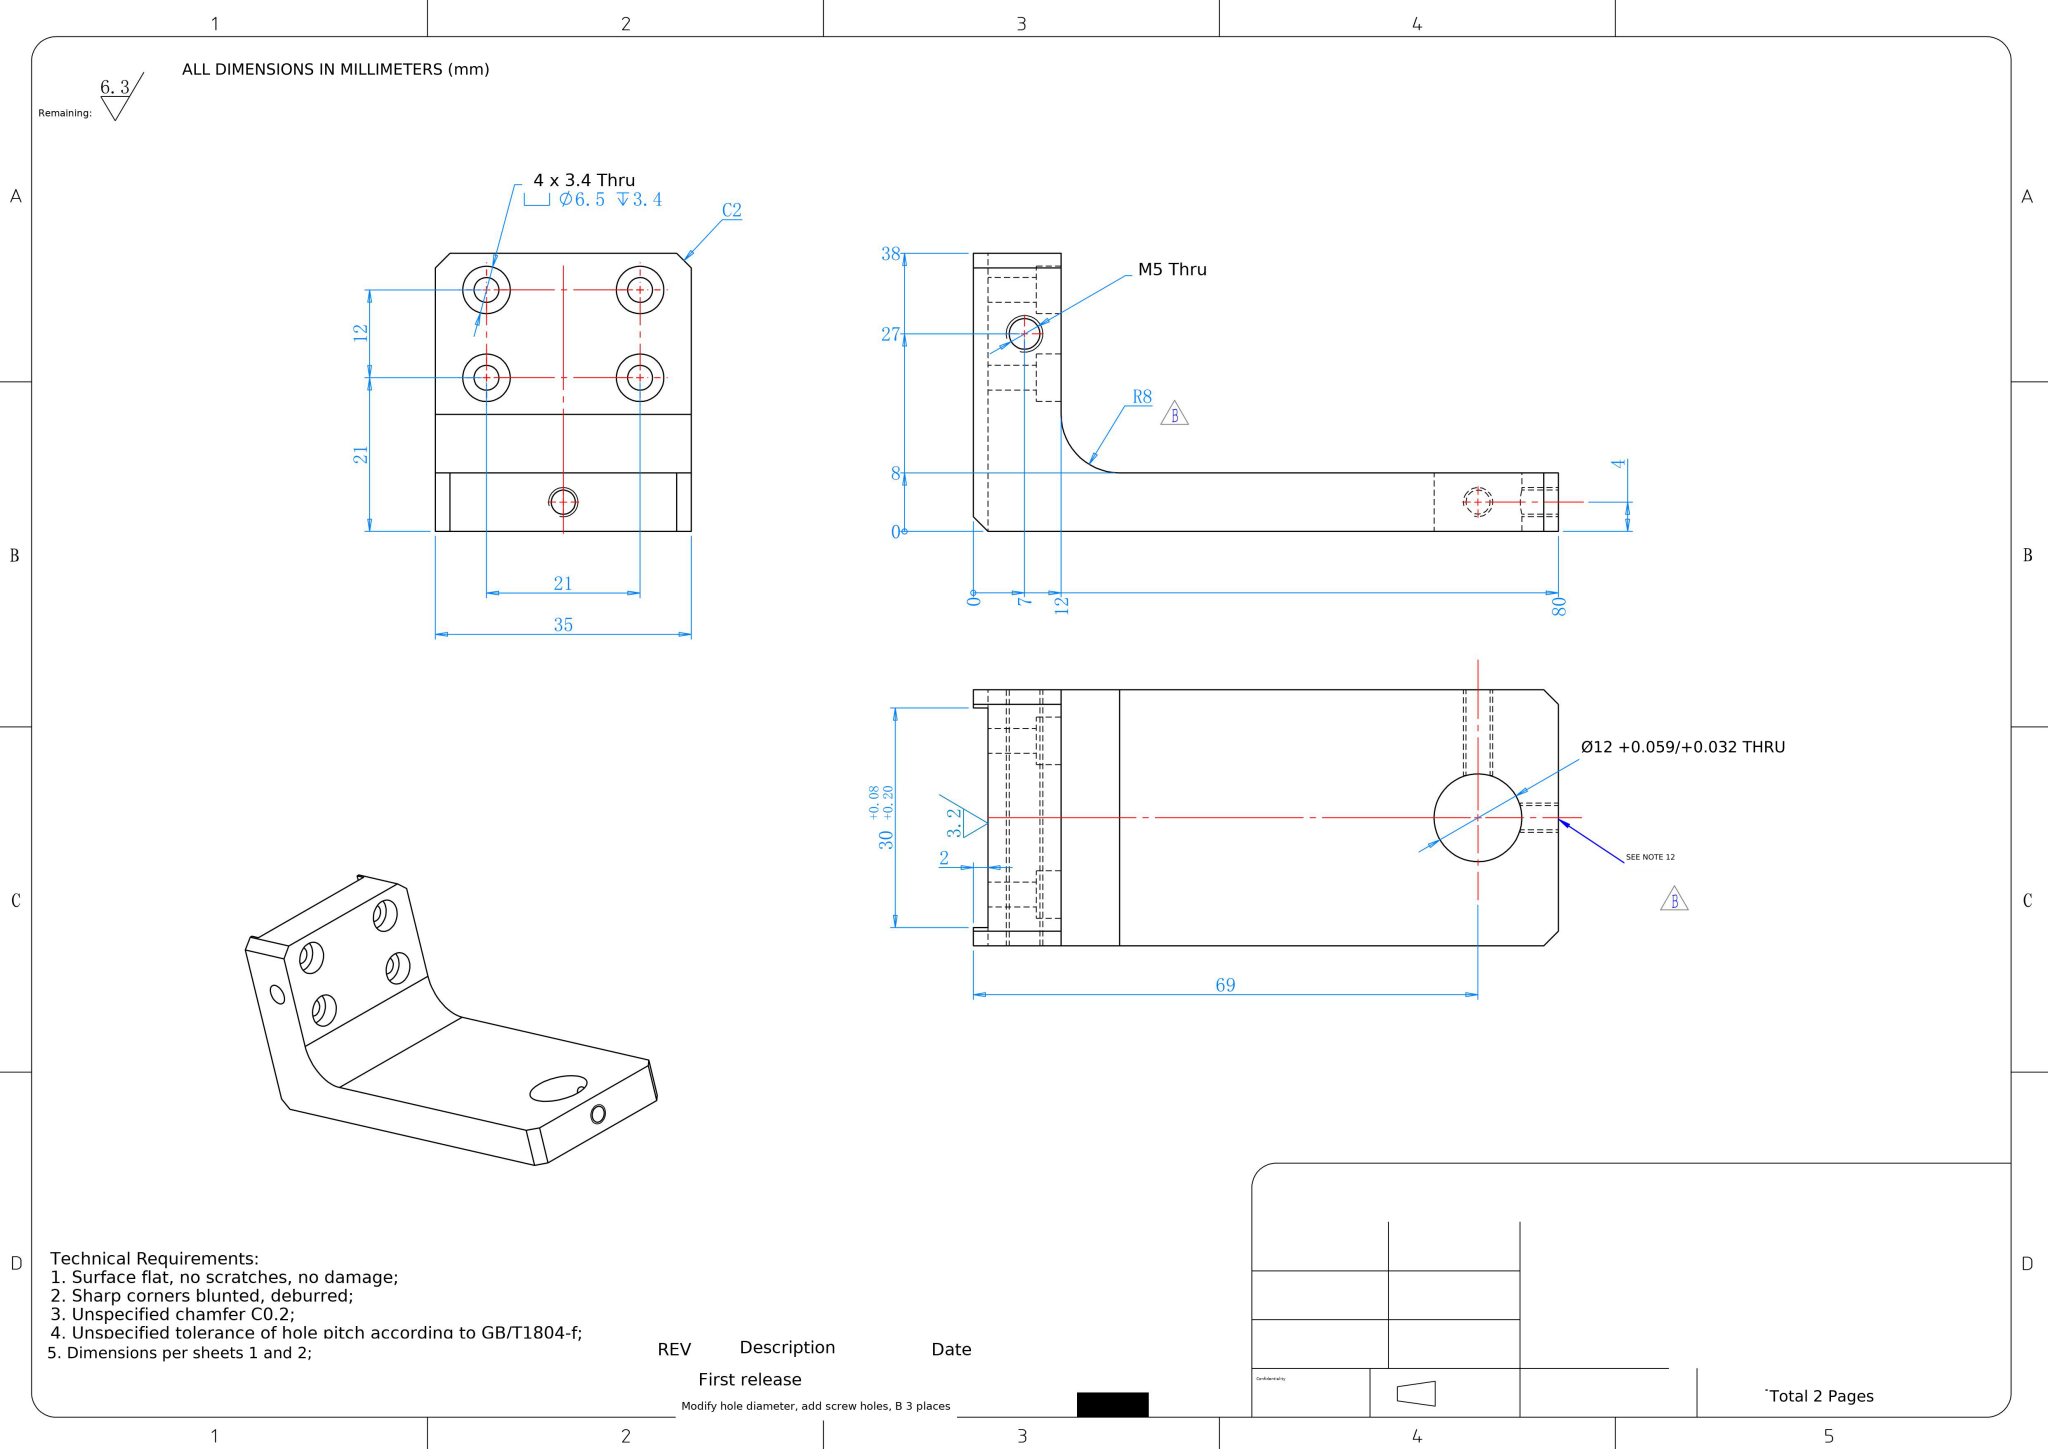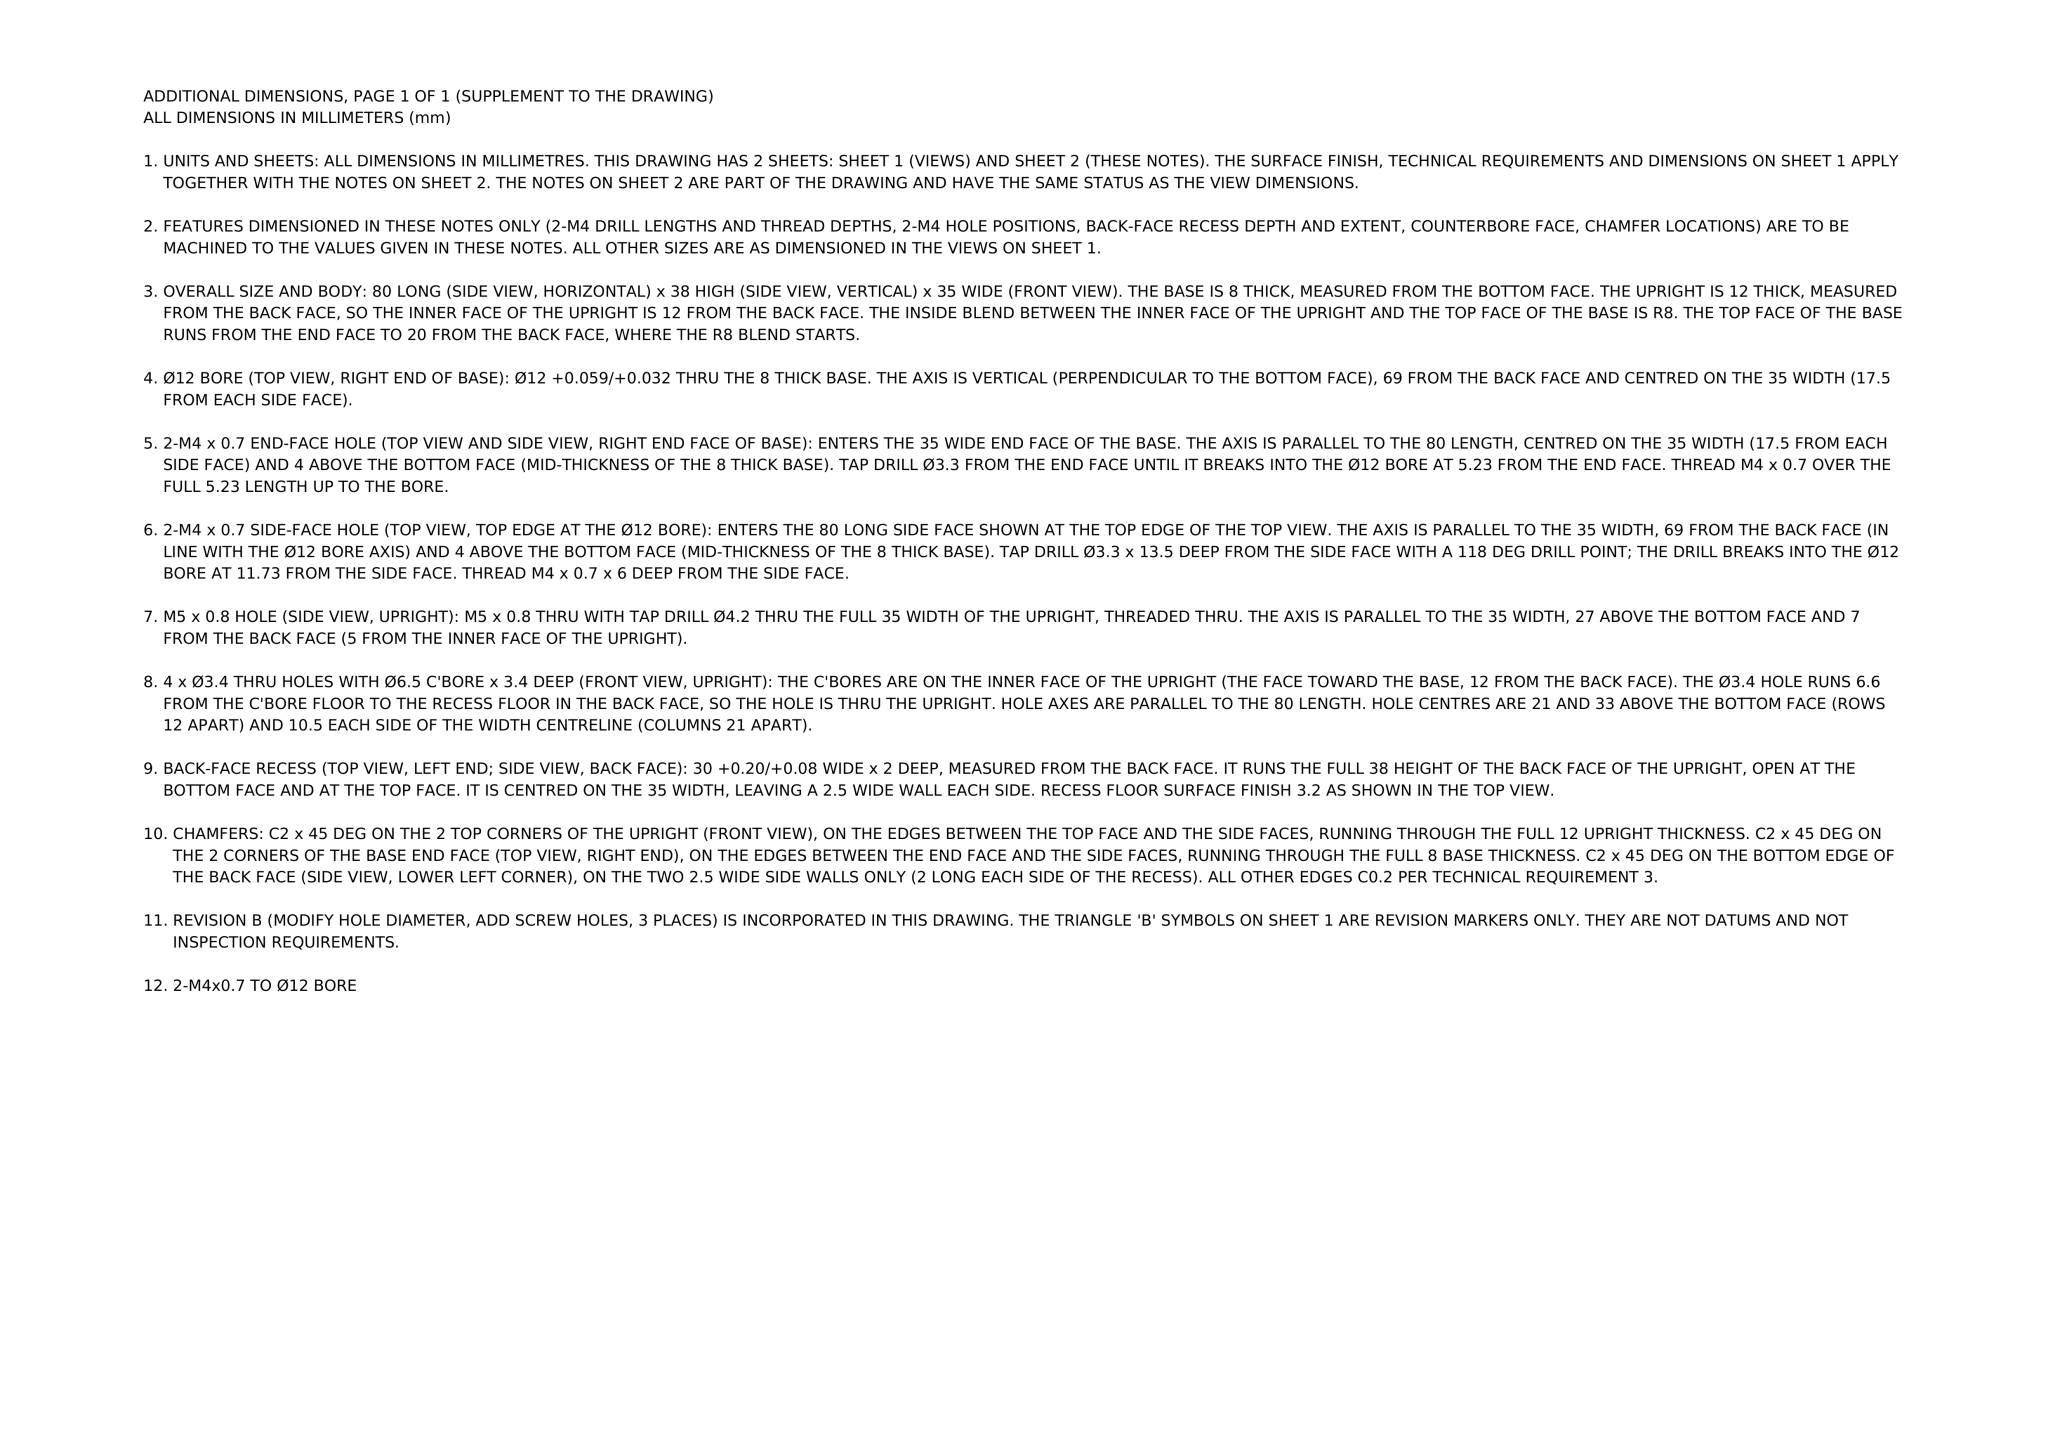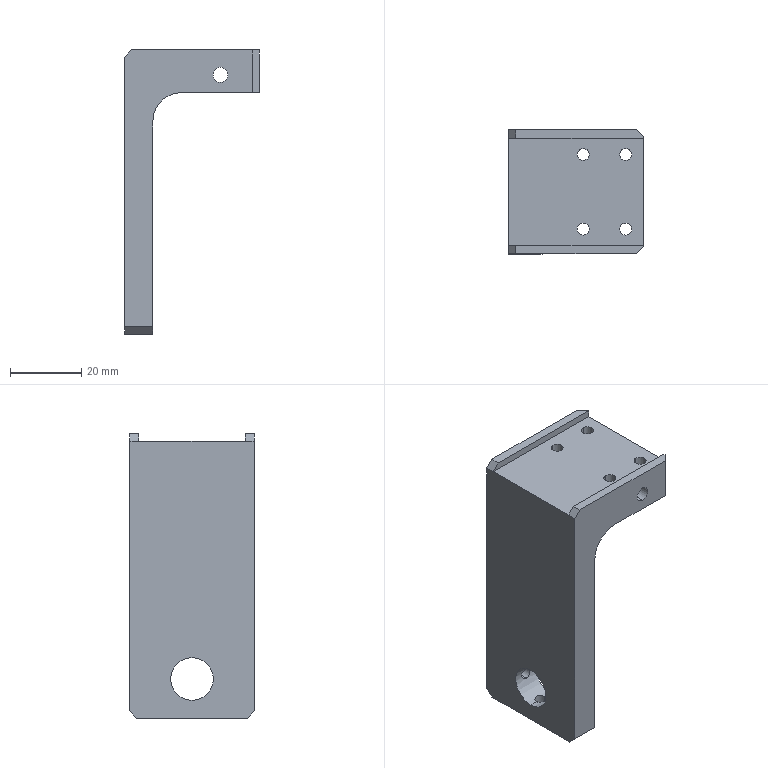Part | NX | mm | 1 solid | 47 faces | box 38 x 35 x 80 mm | volume 30888 mm3 | cylinder 25 | plane 22 | commonest cylinder face diameters 6.5 x8 3.4 x8 3.3 x4 4.2 x2 12 x2 16 x1